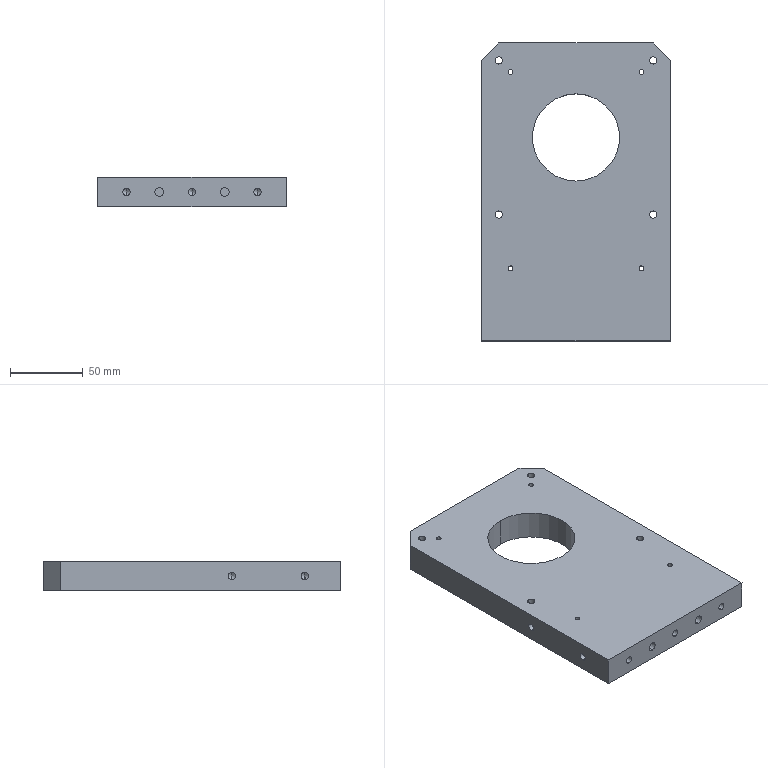Component | SolidWorks | V1ZHXTRotatingPlatformFixingPlateSB1-1 | 1 solid | 68 faces | box 130 x 205 x 20 mm | volume 467729 mm3 | cylinder 40 | cone 18 | plane 10 | commonest cylinder face diameters 5 x26 3.3 x8 6 x4 60 x2 | material 6061-O (SS)
build123d program:
from build123d import *

# Parameters (mm, degrees)
SKETCH1_W             = 280
SKETCH1_H             = 130
BOSS_EXTRUDE1_DEPTH   = 20
M6_TAPPED_HOLE1_D     = 5
SKETCH4_W             = 75
SKETCH4_H             = 130
CUT_EXTRUDE1_DEPTH    = 156.644
M6_TAPPED_HOLE2_D     = 5
M6_TAPPED_HOLE2_DEPTH = 18
M6_TAPPED_HOLE2_TIP   = 1.502
M6_TAPPED_HOLE3_D     = 5
M6_TAPPED_HOLE3_DEPTH = 11
M6_TAPPED_HOLE3_TIP   = 1.502
CHAMFER1_SIZE         = 12
SKETCH14_R            = 30
CUT_EXTRUDE2_DEPTH    = 156.644
SKETCH15_R            = 3
CUT_EXTRUDE3_DEPTH    = 15
M6_TAPPED_HOLE4_D     = 5
M6_TAPPED_HOLE4_DEPTH = 15
M6_TAPPED_HOLE4_TIP   = 1.502
M4_TAPPED_HOLE1_D     = 3.3


with BuildPart() as part:
    # Sketch1 → Boss-Extrude1 (new body)
    with BuildSketch(Plane.XY):
        Rectangle(SKETCH1_W, SKETCH1_H)
    extrude(amount=BOSS_EXTRUDE1_DEPTH)

    # M6 Tapped Hole1 (through all)
    with Locations(Plane.XY.offset(20)):
        with Locations((-53.033, 53.033), (53.033, 53.033), (53.033, -53.033), (-53.033, -53.033)):
            Hole(M6_TAPPED_HOLE1_D / 2)

    # Sketch4 → Cut-Extrude1 (cut, through all)
    with BuildSketch(Plane.XY.offset(20)):
        with Locations((-102.5, 0)):
            Rectangle(SKETCH4_W, SKETCH4_H)
    extrude(amount=-CUT_EXTRUDE1_DEPTH, mode=Mode.SUBTRACT)

    # M6 Tapped Hole2
    with Locations(Plane(origin=(0, -65, 0), x_dir=(-1, 0, 0), z_dir=(0, -1, 0))):
        with Locations((-115, -10), (-65, -10), (-15, -10), (35, -10)):
            Hole(M6_TAPPED_HOLE2_D / 2, depth=M6_TAPPED_HOLE2_DEPTH)
            with Locations((0, 0, -(M6_TAPPED_HOLE2_DEPTH + M6_TAPPED_HOLE2_TIP / 2))):  # 118° drill point
                Cone(0, M6_TAPPED_HOLE2_D / 2, M6_TAPPED_HOLE2_TIP, mode=Mode.SUBTRACT)

    # M6 Tapped Hole3
    with Locations(Plane(origin=(140, 0, 0), x_dir=(0, 0, -1), z_dir=(1, 0, 0))):
        with Locations((-10, 45), (-10, 0), (-10, -45)):
            Hole(M6_TAPPED_HOLE3_D / 2, depth=M6_TAPPED_HOLE3_DEPTH)
            with Locations((0, 0, -(M6_TAPPED_HOLE3_DEPTH + M6_TAPPED_HOLE3_TIP / 2))):  # 118° drill point
                Cone(0, M6_TAPPED_HOLE3_D / 2, M6_TAPPED_HOLE3_TIP, mode=Mode.SUBTRACT)

    # Chamfer1
    chamfer1_edges = [part.edges().sort_by_distance(p)[0] for p in [
        (-65, 65, 10),
        (-65, -65, 10),
    ]]
    chamfer(chamfer1_edges, length=CHAMFER1_SIZE)

    # Sketch14 → Cut-Extrude2 (cut, through all)
    with BuildSketch(Plane.XY.offset(20)):
        Circle(SKETCH14_R)
    extrude(amount=-CUT_EXTRUDE2_DEPTH, mode=Mode.SUBTRACT)

    # Sketch15 → Cut-Extrude3 (cut)
    with BuildSketch(Plane(origin=(140, 0, 0), x_dir=(0, 0, -1), z_dir=(1, 0, 0))):
        with Locations((-10, -22.5)):
            Circle(SKETCH15_R)
        with Locations((-10, 22.5)):
            Circle(SKETCH15_R)
    extrude(amount=-CUT_EXTRUDE3_DEPTH, mode=Mode.SUBTRACT)

    # M6 Tapped Hole4
    with Locations(Plane(origin=(0, 65, 0), x_dir=(1, 0, 0), z_dir=(0, 1, 0))):
        with Locations((115, -10), (65, -10)):
            Hole(M6_TAPPED_HOLE4_D / 2, depth=M6_TAPPED_HOLE4_DEPTH)
            with Locations((0, 0, -(M6_TAPPED_HOLE4_DEPTH + M6_TAPPED_HOLE4_TIP / 2))):  # 118° drill point
                Cone(0, M6_TAPPED_HOLE4_D / 2, M6_TAPPED_HOLE4_TIP, mode=Mode.SUBTRACT)

    # M4 Tapped Hole1 (through all)
    with Locations(Plane(origin=(0, 0, 0), x_dir=(-1, 0, 0), z_dir=(0, 0, -1))):
        with Locations((-90, 45), (-90, -45), (45, -45), (45, 45)):
            Hole(M4_TAPPED_HOLE1_D / 2)


solid = part.part

# Placed as in the assembly
solid = solid.moved(Location((176.521, -204.132, 568.739), (180, 0, 90)))